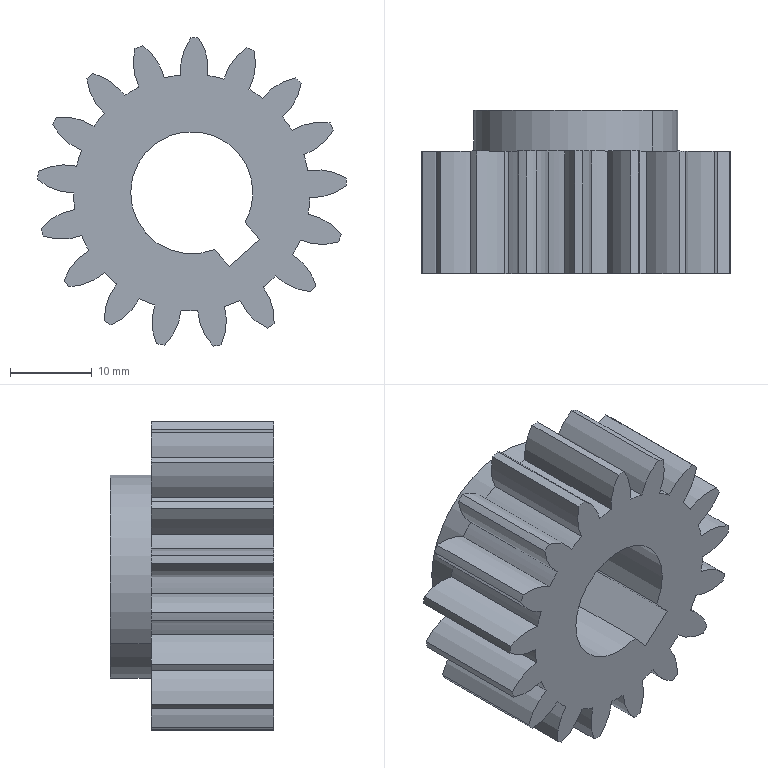Component | SolidWorks | CrankshaftOne-1_spur gear_gb-1 | 1 solid | 83 faces | box 37.91 x 20 x 37.82 mm | volume 11734 mm3 | cylinder 77 | plane 6 | commonest cylinder face diameters 13.6 x38 38 x17 28.998 x17 15 x3 25 x2
build123d program:
from build123d import *

# Parameters (mm, degrees)
BASPROSKE_W      = 15
BASPROSKE_H      = 19
TOOTHCUT_DEPTH   = 31.773
TEETHCUTS_COUNT  = 17
TEETHCUTS_ANGLE  = 338.824
HUBNEAONESKE_R   = 12.5
HUBNEARONE_DEPTH = 5
BORSKE_R         = 7.5
BORE_DEPTH       = 20
KEYSKE_W         = 5
KEYSKE_H         = 9.8
KEYWAY_DEPTH     = 20


with BuildPart() as part:
    # BasProSke → Base-Revolve (revolve)
    with BuildSketch(Plane(origin=(0, 0, 0), x_dir=(1, 0, 0), z_dir=(0, 1, 0)), mode=Mode.PRIVATE) as base_revolve_sk:
        with Locations((7.5, 9.5)):
            Rectangle(BASPROSKE_W, BASPROSKE_H)
    revolve(base_revolve_sk.sketch.rotate(Axis((-10, 0, 0), (1, 0, 0)), 180), axis=Axis((-10, 0, 0), (1, 0, 0)))

    # TooCutSke → ToothCut (cut, through all)
    with BuildSketch(Plane(origin=(0, 0, 0), x_dir=(0, 0, -1), z_dir=(1, 0, 0))):
        with BuildLine():
            ThreePointArc((1.02, 14.463), (0, 14.499), (-1.02, 14.463))
            ThreePointArc((-1.02, 14.463), (-1.633, 16.804), (-3.026, 18.783))
            ThreePointArc((-3.026, 18.783), (0, 19.025), (3.026, 18.783))
            ThreePointArc((3.026, 18.783), (1.633, 16.804), (1.02, 14.463))
        make_face()
    toothcut = extrude(amount=TOOTHCUT_DEPTH, mode=Mode.SUBTRACT)

    # TeethCuts: ToothCut ×17 about axis
    teethcuts_axis = Axis((-10, 0, 0), (1, 0, 0))
    for i in range(1, TEETHCUTS_COUNT):
        add(toothcut.rotate(teethcuts_axis, i * TEETHCUTS_ANGLE / (TEETHCUTS_COUNT - 1)), mode=Mode.SUBTRACT)

    # HubNeaOneSke → HubNearOne (add)
    with BuildSketch(Plane.ZY):
        with Locations(Location((0, 0, 0), (0, 0, 180))):
            Circle(HUBNEAONESKE_R)
    extrude(amount=HUBNEARONE_DEPTH)

    # BorSke → Bore (cut, symmetric)
    with BuildSketch(Plane(origin=(0, 0, 0), x_dir=(0, 0, -1), z_dir=(1, 0, 0))):
        with Locations(Location((0, 0, 0), (0, 0, 180))):
            Circle(BORSKE_R)
    extrude(amount=BORE_DEPTH, both=True, mode=Mode.SUBTRACT)

    # KeySke → Keyway (cut, symmetric)
    with BuildSketch(Plane(origin=(0, 0, 0), x_dir=(0, 0, -1), z_dir=(1, 0, 0))):
        with Locations((0, 4.9)):
            Rectangle(KEYSKE_W, KEYSKE_H)
    extrude(amount=KEYWAY_DEPTH, both=True, mode=Mode.SUBTRACT)


solid = part.part

# Placed as in the assembly
solid = solid.moved(Location((-199.914, 68.266, -166.507), (0, 48.794, -90)))